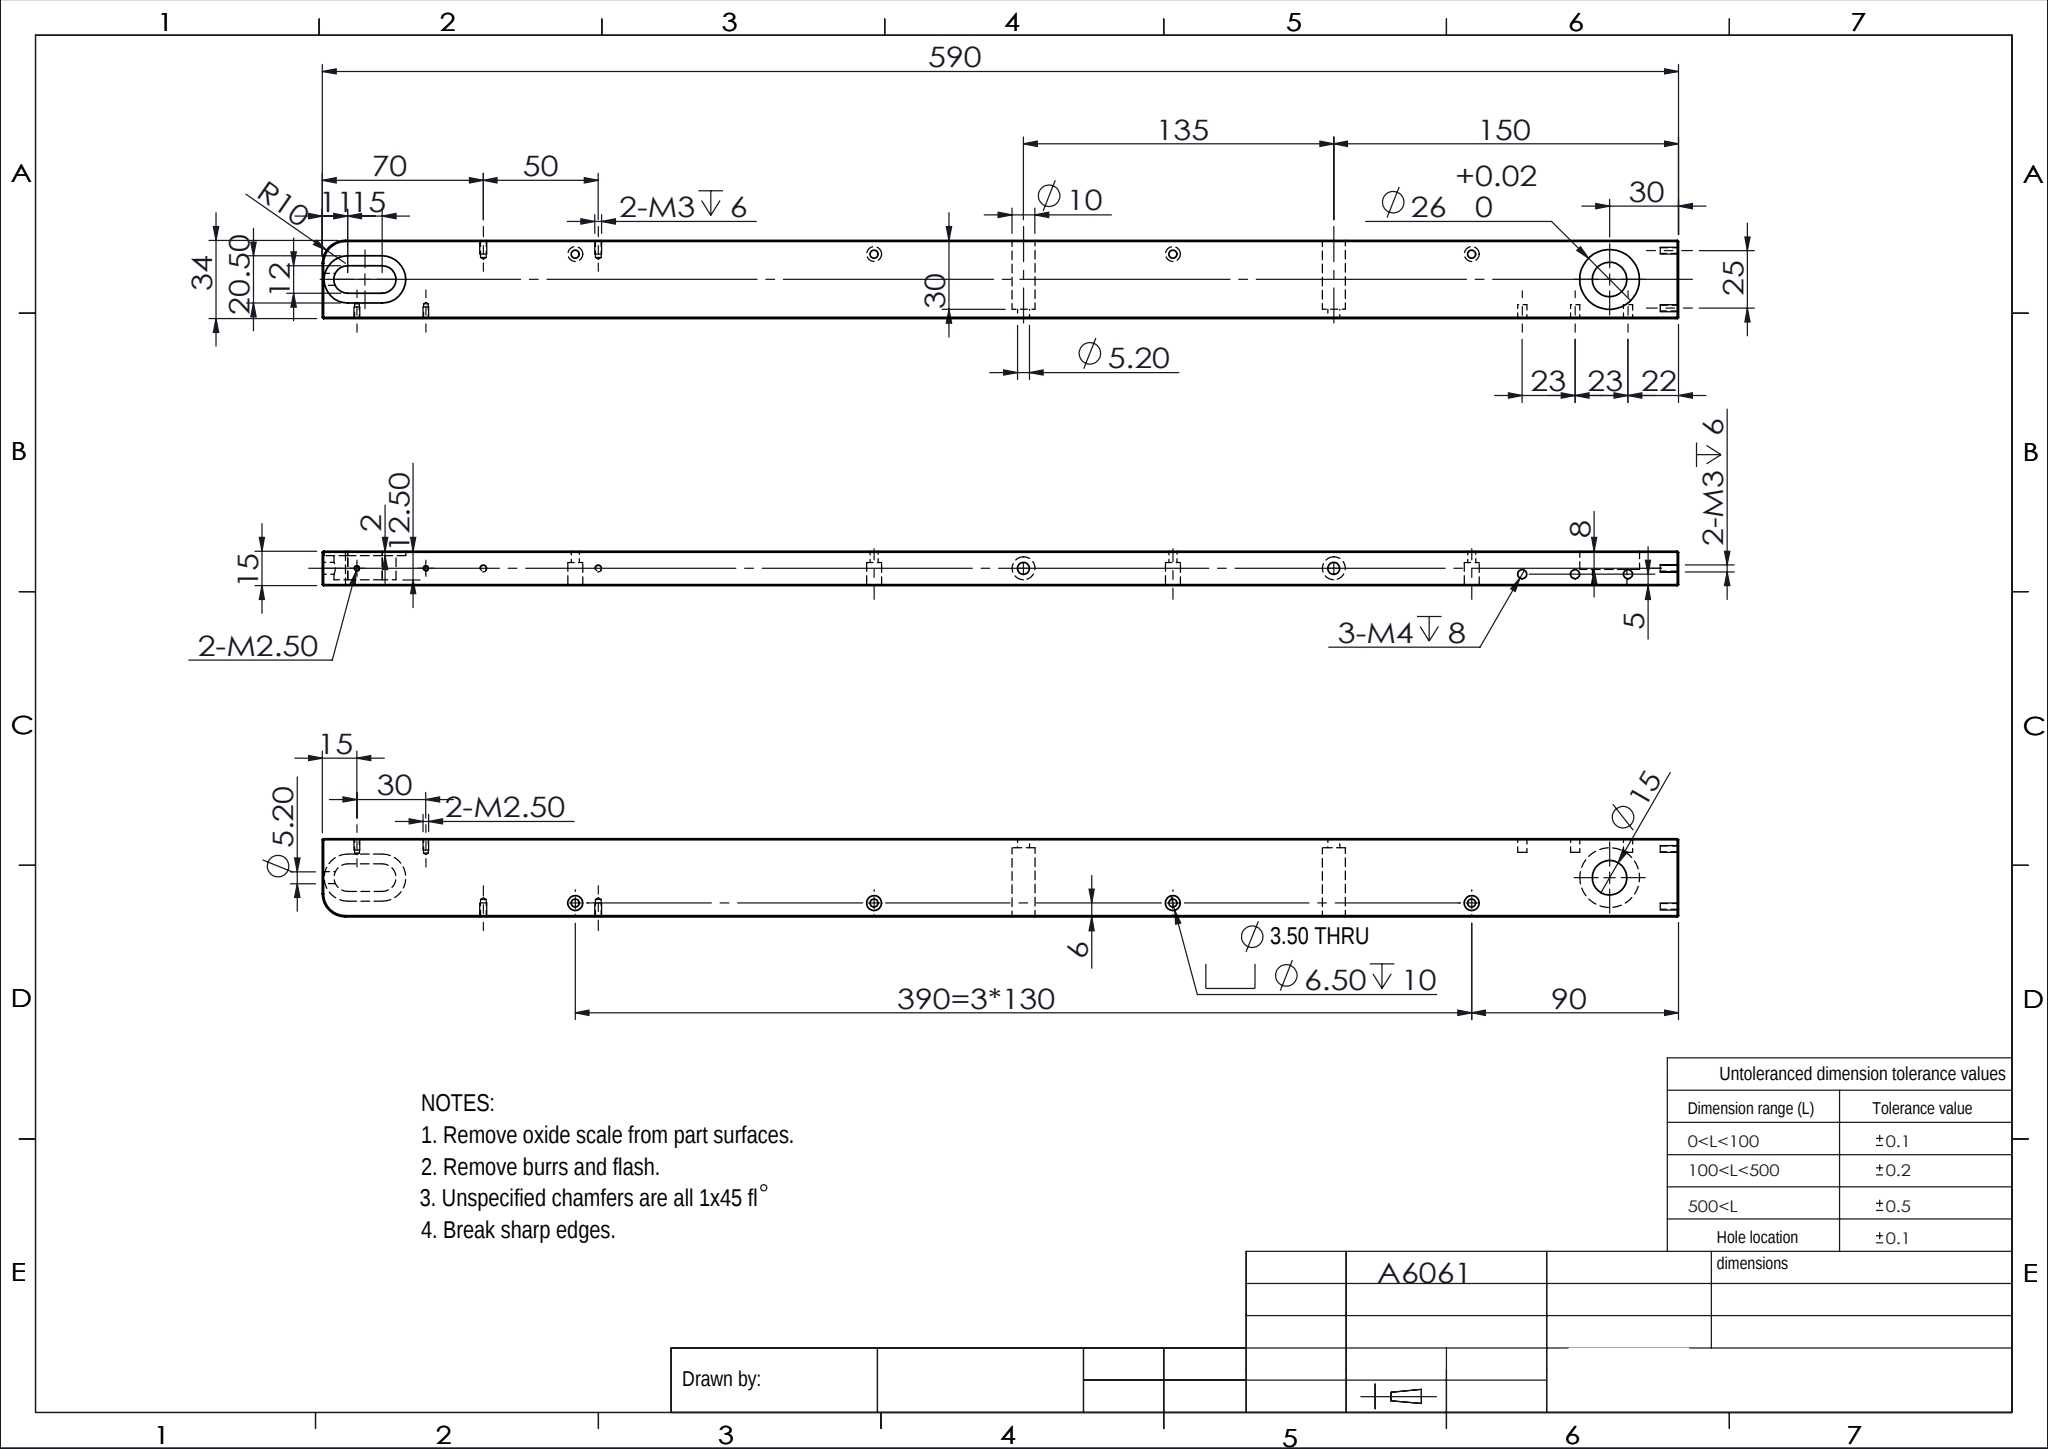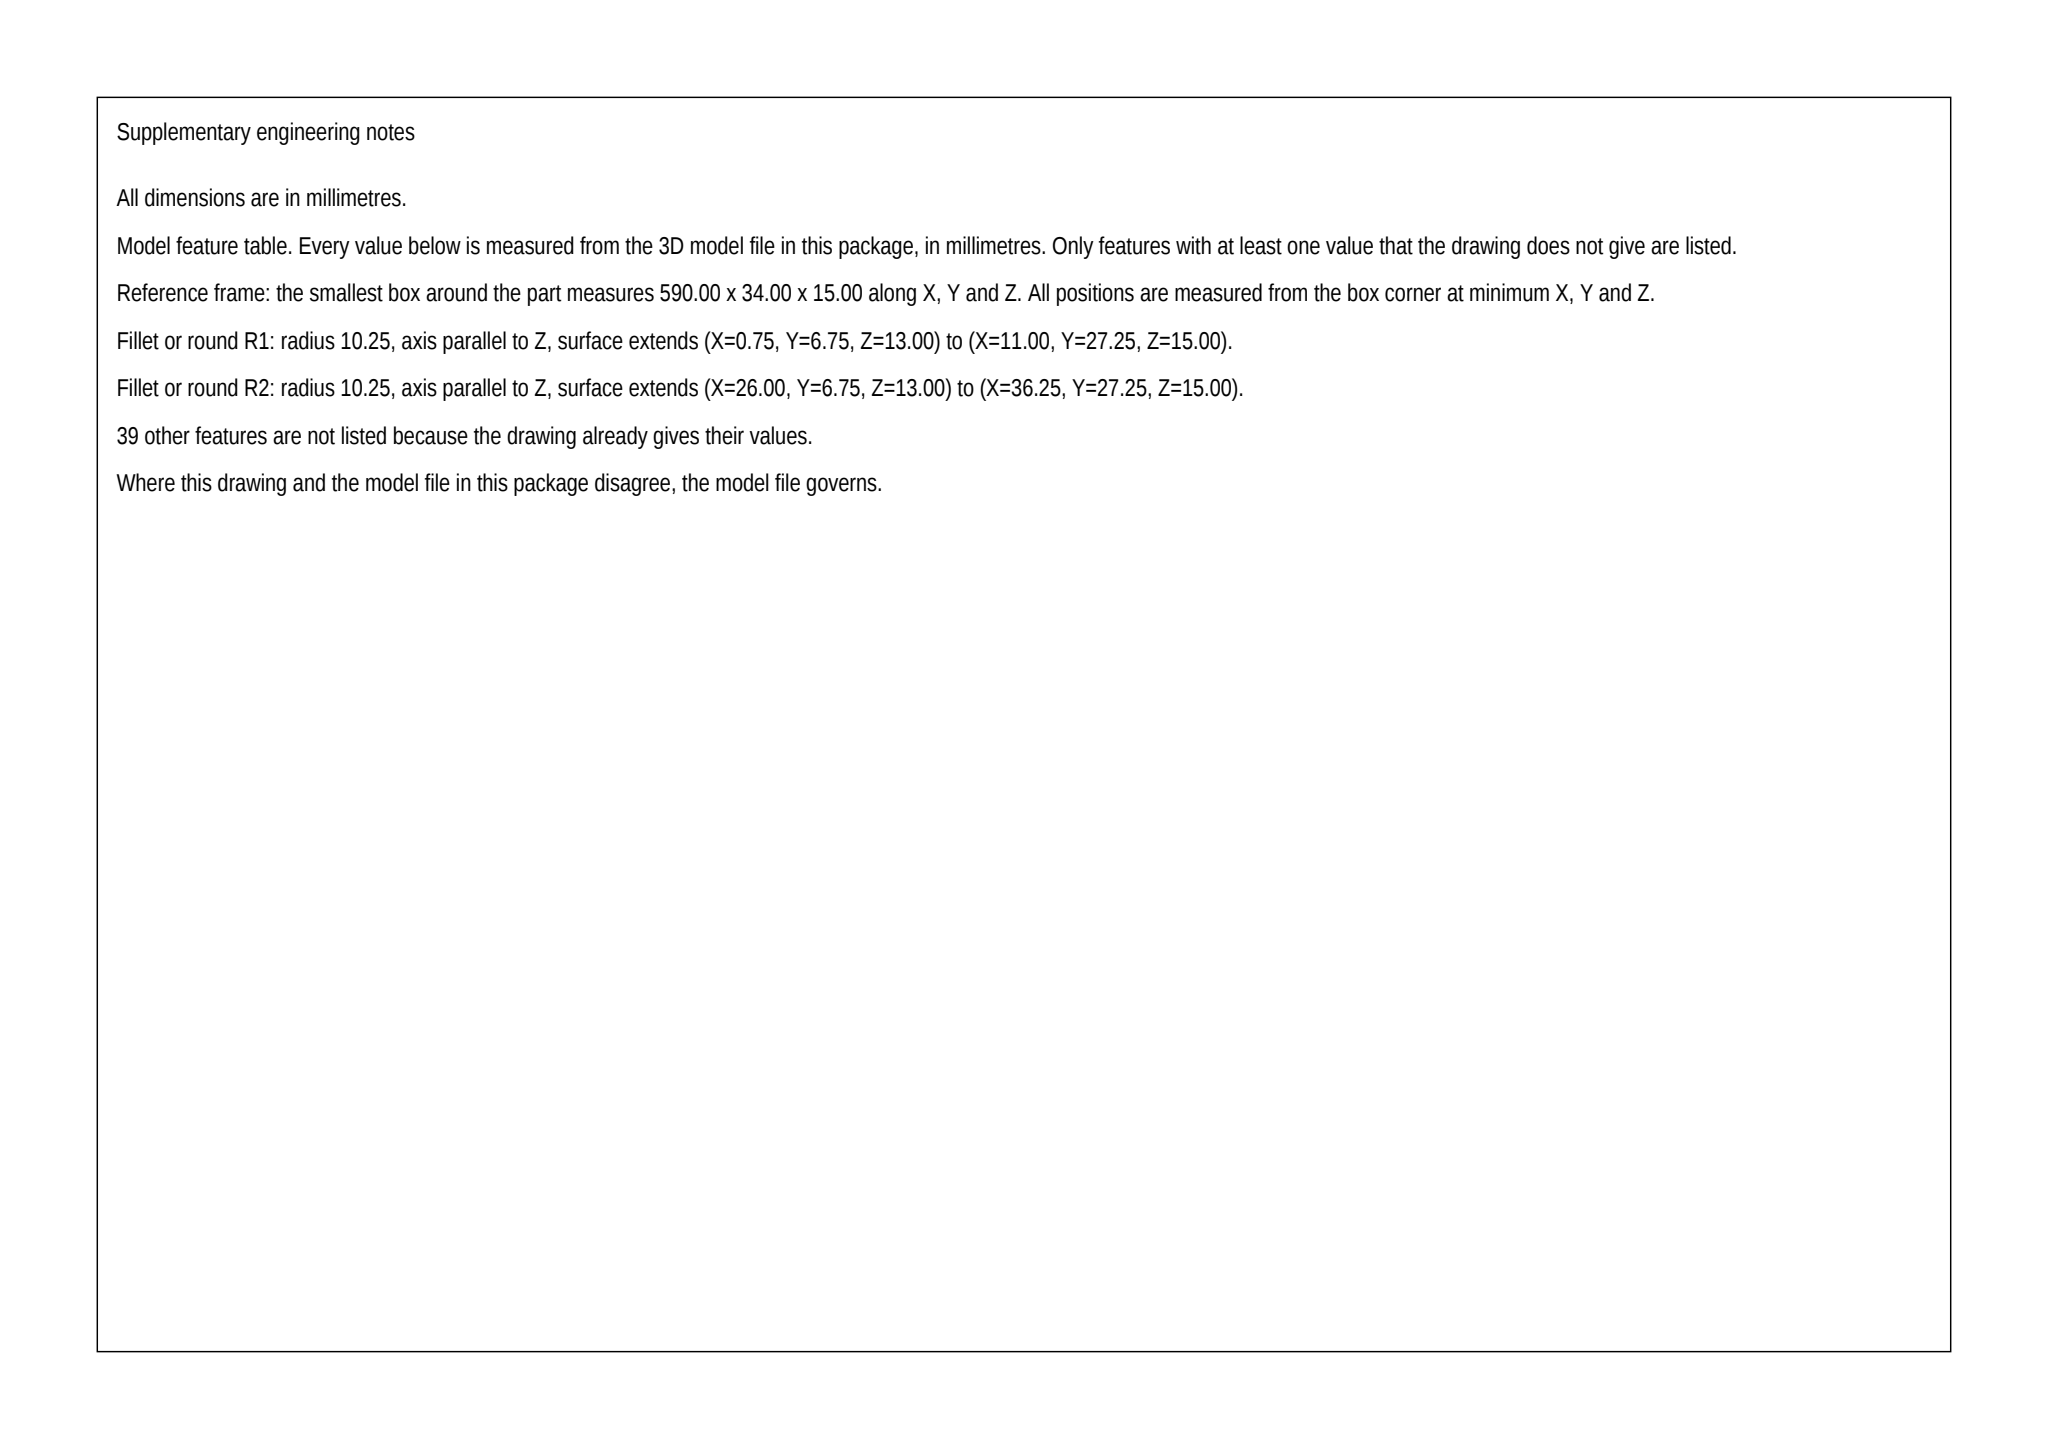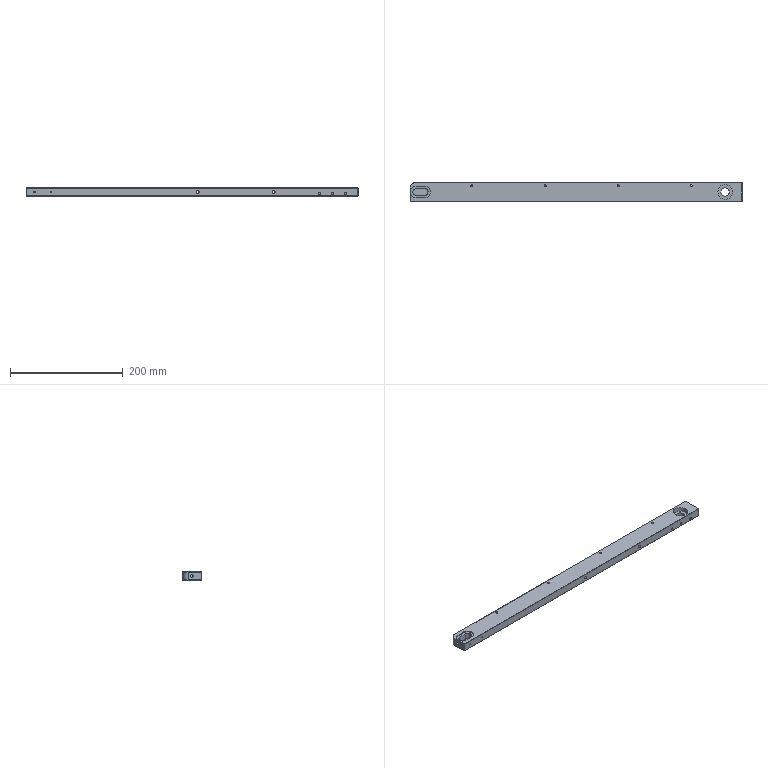Part | SolidWorks | mm | 1 solid | 106 faces | box 590 x 34 x 15 mm | volume 283490 mm3 | cylinder 55 | plane 41 | cone 10 | commonest cylinder face diameters 2.5 x8 6.5 x8 3.5 x8 5.2 x6 4 x6 10 x4 2.05 x4 12 x3
Drawing notes:
SLOT 12 WIDE x 27 OAL DP 10.5, CTRS 11 & 26 FM LH END, ON Y CL 17 | from the solid: cyl Ø12 axis z @ (11,17) & (26,17) L=10.5; ctr dist 15, OAL 15+12=27; y17=mid of 34
SLOT CBORE 20.5 WIDE x 35.5 OAL DP 2, COAX W/ SLOT | from the solid: cyl Ø20.5 axis z @ (11,17) & (26,17) L=2.0; 15+20.5=35.5
Ø5.20 IN LH END FACE DP 5.59, Z CL 7.5, BREAKS INTO SLOT | from the solid: cyl [5.2,'x',[null,17.0,7.5],5.59] from x=0 face; slot Ø12 dp 10.5 at x=11/26
2-M2.5 DP 6.35 IN SIDE FACE (NOT BOT), Z CL 7.5, AT 15 & 45 FM LH END | from the solid: cyl Ø2.05 axis y @ x=15 & 45, z=7.5, L=6.35 (M2.5 tap drill); cone 118° ref dia 2.05
Ø5.20 THRU W/ Ø10 CBORE DP 30: CLS 305 & 440 FM LH END FACE | from the solid: cyl Ø10 axis y @ x=305,440 z=7.5 L=30; Ø5.2 axis y same x L=4; 440-305=135, 590-440=150
Ø26 +0.02/0 CBORE DP 8 FM TOP, CL 30 FM RH END | from the solid: cyl Ø26 axis z @ (560,17) L=8; bbox x=590 -> 590-560=30
Ø15 UNDER Ø26 DP 7, BREAKS THRU BOT FACE; CSK Ø19 x 90° AT BOT | from the solid: cyl Ø15 axis z @ (560,17) L=7; 8+7=15=thk, planes z=0/z=15; cones[90.0,19.0] x2
2-M3 DP 6 (DRILL DP 8) IN RH END FACE, 25 APART SYMM, Z CL 7.5 | from the solid: cyl Ø2.5 axis x @ y=4.5 & 29.5, z=7.5, L=8 fm x=590; 29.5-4.5=25 symm abt y=17
3-M4 DP 8 IN SIDE FACE AT 22, 45, 68 FM RH END, AXES 5 FM BOT FACE | from the solid: cyl Ø4.0 axis y @ x=522,545,568, z=5.0, L=6; 590-568=22, 590-545=45, 590-522=68
ALL UNSPEC CHAMFERS C1 (1x45°); BLUNT SHARP CORNERS | from the solid: sheet note text corrupted '1x454'; no fillet radii in model